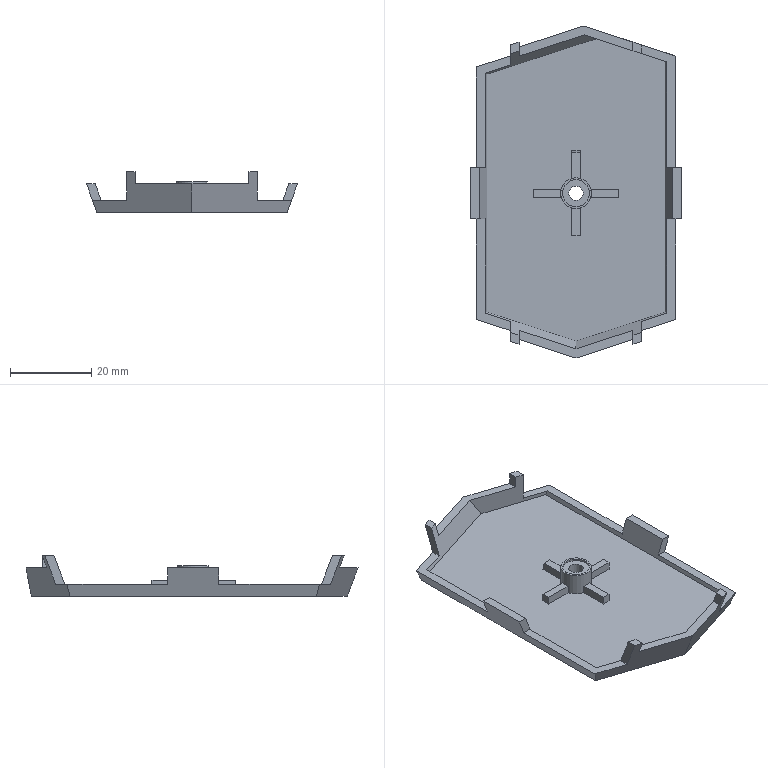Component | NX | COVER_PLATE | 5 solids | 67 faces | volume 8233 mm3 | plane 63 | cylinder 4 | commonest cylinder face diameters 7.54 x2 3.5 x1 6.6 x1